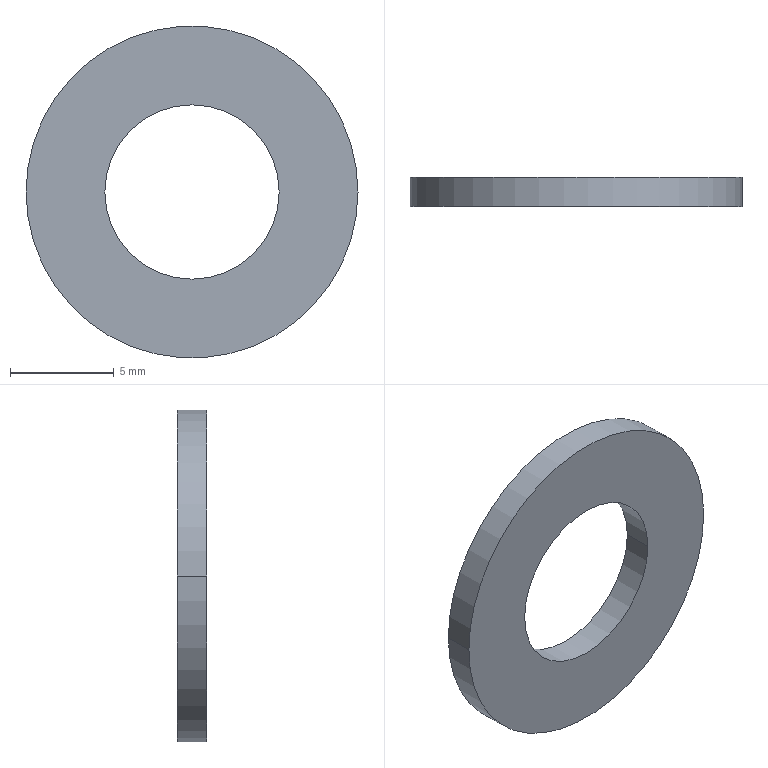Component | SolidWorks | FlatWasher_8-1 | 1 solid | 6 faces | box 16 x 1.4 x 16 mm | volume 204 mm3 | cylinder 4 | plane 2 | commonest cylinder face diameters 8.4 x2 16 x2 | material Plain Carbon Steel
build123d program:
from build123d import *

# Parameters (mm, degrees)
SKETCH1_R           = 8
SKETCH1_R_2         = 4.2
BOSS_EXTRUDE1_DEPTH = 1.4


with BuildPart() as part:
    # Sketch1 → Boss-Extrude1 (new body)
    with BuildSketch(Plane.XY):
        Circle(SKETCH1_R)
        Circle(SKETCH1_R_2, mode=Mode.SUBTRACT)
    extrude(amount=BOSS_EXTRUDE1_DEPTH)


solid = part.part

# Placed as in the assembly
solid = solid.moved(Location((29.475, -68.5, 229.781), (90, 0, 0)))
STEP:
#1=CARTESIAN_POINT('',(0.9951,-2.752,9.046));
#2=VERTEX_POINT('',#1);
#3=CARTESIAN_POINT('',(1.326,-2.752,9.046));
#4=VERTEX_POINT('',#3);
#5=CARTESIAN_POINT('',(1.16,-2.752,9.046));
#6=DIRECTION('',(0.,-1.,0.));
#7=DIRECTION('',(1.,0.,0.));
#8=AXIS2_PLACEMENT_3D('',#5,#6,#7);
#9=CIRCLE('',#8,0.1654);
#10=EDGE_CURVE('',#2,#4,#9,.T.);
#11=ORIENTED_EDGE('',*,*,#10,.T.);
#12=CARTESIAN_POINT('',(1.326,-2.697,9.046));
#13=VERTEX_POINT('',#12);
#14=CARTESIAN_POINT('',(1.326,-2.752,9.046));
#15=DIRECTION('',(-0.,1.,-0.));
#16=VECTOR('',#15,39.37);
#17=LINE('',#14,#16);
#18=EDGE_CURVE('',#4,#13,#17,.T.);
#19=ORIENTED_EDGE('',*,*,#18,.T.);
#20=CARTESIAN_POINT('',(0.9951,-2.697,9.046));
#21=VERTEX_POINT('',#20);
#22=CARTESIAN_POINT('',(1.16,-2.697,9.046));
#23=DIRECTION('',(0.,-1.,0.));
#24=DIRECTION('',(1.,0.,0.));
#25=AXIS2_PLACEMENT_3D('',#22,#23,#24);
#26=CIRCLE('',#25,0.1654);
#27=EDGE_CURVE('',#21,#13,#26,.T.);
#28=ORIENTED_EDGE('',*,*,#27,.F.);
#29=CARTESIAN_POINT('',(0.9951,-2.752,9.046));
#30=DIRECTION('',(-0.,1.,-0.));
#31=VECTOR('',#30,39.37);
#32=LINE('',#29,#31);
#33=EDGE_CURVE('',#2,#21,#32,.T.);
#34=ORIENTED_EDGE('',*,*,#33,.F.);
#35=EDGE_LOOP('',(#11,#19,#28,#34));
#36=FACE_OUTER_BOUND('',#35,.T.);
#37=CARTESIAN_POINT('',(1.16,-2.752,9.046));
#38=DIRECTION('',(-0.,1.,-0.));
#39=DIRECTION('',(-1.,0.,0.));
#40=AXIS2_PLACEMENT_3D('',#37,#38,#39);
#41=CYLINDRICAL_SURFACE('',#40,0.1654);
#42=ADVANCED_FACE('',(#36),#41,.F.);
#43=CARTESIAN_POINT('',(1.475,-2.752,9.046));
#44=VERTEX_POINT('',#43);
#45=CARTESIAN_POINT('',(0.8455,-2.752,9.046));
#46=VERTEX_POINT('',#45);
#47=CARTESIAN_POINT('',(1.16,-2.752,9.046));
#48=DIRECTION('',(0.,-1.,0.));
#49=DIRECTION('',(1.,0.,0.));
#50=AXIS2_PLACEMENT_3D('',#47,#48,#49);
#51=CIRCLE('',#50,0.315);
#52=EDGE_CURVE('',#44,#46,#51,.T.);
#53=ORIENTED_EDGE('',*,*,#52,.F.);
#54=CARTESIAN_POINT('',(1.475,-2.697,9.046));
#55=VERTEX_POINT('',#54);
#56=CARTESIAN_POINT('',(1.475,-2.752,9.046));
#57=DIRECTION('',(-0.,1.,-0.));
#58=VECTOR('',#57,39.37);
#59=LINE('',#56,#58);
#60=EDGE_CURVE('',#44,#55,#59,.T.);
#61=ORIENTED_EDGE('',*,*,#60,.T.);
#62=CARTESIAN_POINT('',(0.8455,-2.697,9.046));
#63=VERTEX_POINT('',#62);
#64=CARTESIAN_POINT('',(1.16,-2.697,9.046));
#65=DIRECTION('',(0.,-1.,0.));
#66=DIRECTION('',(1.,0.,0.));
#67=AXIS2_PLACEMENT_3D('',#64,#65,#66);
#68=CIRCLE('',#67,0.315);
#69=EDGE_CURVE('',#55,#63,#68,.T.);
#70=ORIENTED_EDGE('',*,*,#69,.T.);
#71=CARTESIAN_POINT('',(0.8455,-2.752,9.046));
#72=DIRECTION('',(-0.,1.,-0.));
#73=VECTOR('',#72,39.37);
#74=LINE('',#71,#73);
#75=EDGE_CURVE('',#46,#63,#74,.T.);
#76=ORIENTED_EDGE('',*,*,#75,.F.);
#77=EDGE_LOOP('',(#53,#61,#70,#76));
#78=FACE_OUTER_BOUND('',#77,.T.);
#79=CARTESIAN_POINT('',(1.16,-2.752,9.046));
#80=DIRECTION('',(-0.,1.,-0.));
#81=DIRECTION('',(-1.,0.,0.));
#82=AXIS2_PLACEMENT_3D('',#79,#80,#81);
#83=CYLINDRICAL_SURFACE('',#82,0.315);
#84=ADVANCED_FACE('',(#78),#83,.T.);
#85=CARTESIAN_POINT('',(1.16,-2.752,9.046));
#86=DIRECTION('',(0.,-1.,0.));
#87=DIRECTION('',(1.,0.,0.));
#88=AXIS2_PLACEMENT_3D('',#85,#86,#87);
#89=CIRCLE('',#88,0.315);
#90=EDGE_CURVE('',#46,#44,#89,.T.);
#91=ORIENTED_EDGE('',*,*,#90,.T.);
#92=ORIENTED_EDGE('',*,*,#52,.T.);
#93=EDGE_LOOP('',(#91,#92));
#94=FACE_OUTER_BOUND('',#93,.T.);
#95=ORIENTED_EDGE('',*,*,#10,.F.);
#96=CARTESIAN_POINT('',(1.16,-2.752,9.046));
#97=DIRECTION('',(0.,-1.,0.));
#98=DIRECTION('',(1.,0.,0.));
#99=AXIS2_PLACEMENT_3D('',#96,#97,#98);
#100=CIRCLE('',#99,0.1654);
#101=EDGE_CURVE('',#4,#2,#100,.T.);
#102=ORIENTED_EDGE('',*,*,#101,.F.);
#103=EDGE_LOOP('',(#95,#102));
#104=FACE_BOUND('',#103,.T.);
#105=CARTESIAN_POINT('',(1.16,-2.752,9.046));
#106=DIRECTION('',(0.,-1.,0.));
#107=DIRECTION('',(1.,0.,-0.));
#108=AXIS2_PLACEMENT_3D('',#105,#106,#107);
#109=PLANE('',#108);
#110=ADVANCED_FACE('',(#94,#104),#109,.T.);
#111=CARTESIAN_POINT('',(1.16,-2.697,9.046));
#112=DIRECTION('',(0.,-1.,0.));
#113=DIRECTION('',(1.,0.,0.));
#114=AXIS2_PLACEMENT_3D('',#111,#112,#113);
#115=CIRCLE('',#114,0.315);
#116=EDGE_CURVE('',#63,#55,#115,.T.);
#117=ORIENTED_EDGE('',*,*,#116,.F.);
#118=ORIENTED_EDGE('',*,*,#69,.F.);
#119=EDGE_LOOP('',(#117,#118));
#120=FACE_OUTER_BOUND('',#119,.T.);
#121=ORIENTED_EDGE('',*,*,#27,.T.);
#122=CARTESIAN_POINT('',(1.16,-2.697,9.046));
#123=DIRECTION('',(0.,-1.,0.));
#124=DIRECTION('',(1.,0.,0.));
#125=AXIS2_PLACEMENT_3D('',#122,#123,#124);
#126=CIRCLE('',#125,0.1654);
#127=EDGE_CURVE('',#13,#21,#126,.T.);
#128=ORIENTED_EDGE('',*,*,#127,.T.);
#129=EDGE_LOOP('',(#121,#128));
#130=FACE_BOUND('',#129,.T.);
#131=CARTESIAN_POINT('',(1.16,-2.697,9.046));
#132=DIRECTION('',(0.,-1.,0.));
#133=DIRECTION('',(1.,0.,-0.));
#134=AXIS2_PLACEMENT_3D('',#131,#132,#133);
#135=PLANE('',#134);
#136=ADVANCED_FACE('',(#120,#130),#135,.F.);
#137=ORIENTED_EDGE('',*,*,#60,.F.);
#138=ORIENTED_EDGE('',*,*,#90,.F.);
#139=ORIENTED_EDGE('',*,*,#75,.T.);
#140=ORIENTED_EDGE('',*,*,#116,.T.);
#141=EDGE_LOOP('',(#137,#138,#139,#140));
#142=FACE_OUTER_BOUND('',#141,.T.);
#143=CARTESIAN_POINT('',(1.16,-2.752,9.046));
#144=DIRECTION('',(-0.,1.,-0.));
#145=DIRECTION('',(-1.,0.,0.));
#146=AXIS2_PLACEMENT_3D('',#143,#144,#145);
#147=CYLINDRICAL_SURFACE('',#146,0.315);
#148=ADVANCED_FACE('',(#142),#147,.T.);
#149=ORIENTED_EDGE('',*,*,#18,.F.);
#150=ORIENTED_EDGE('',*,*,#101,.T.);
#151=ORIENTED_EDGE('',*,*,#33,.T.);
#152=ORIENTED_EDGE('',*,*,#127,.F.);
#153=EDGE_LOOP('',(#149,#150,#151,#152));
#154=FACE_OUTER_BOUND('',#153,.T.);
#155=CARTESIAN_POINT('',(1.16,-2.752,9.046));
#156=DIRECTION('',(-0.,1.,-0.));
#157=DIRECTION('',(-1.,0.,0.));
#158=AXIS2_PLACEMENT_3D('',#155,#156,#157);
#159=CYLINDRICAL_SURFACE('',#158,0.1654);
#160=ADVANCED_FACE('',(#154),#159,.F.);
#161=CLOSED_SHELL('',(#42,#84,#110,#136,#148,#160));
#162=MANIFOLD_SOLID_BREP('',#161);
#163=CARTESIAN_POINT('',(0.,0.,0.));
#164=DIRECTION('',(0.,0.,1.));
#165=DIRECTION('',(1.,0.,0.));
#166=AXIS2_PLACEMENT_3D('',#163,#164,#165);
#167=(LENGTH_UNIT()NAMED_UNIT(*)SI_UNIT($,.METRE.));
#168=LENGTH_MEASURE_WITH_UNIT(LENGTH_MEASURE(0.0254),#167);
#169=DIMENSIONAL_EXPONENTS(1.,0.,0.,0.,0.,0.,0.);
#170=(CONVERSION_BASED_UNIT('',#168)LENGTH_UNIT()NAMED_UNIT(#169));
#171=UNCERTAINTY_MEASURE_WITH_UNIT(LENGTH_MEASURE(0.00001),#170,'','');
#172=(NAMED_UNIT(*)PLANE_ANGLE_UNIT()SI_UNIT($,.RADIAN.));
#173=(NAMED_UNIT(*)SI_UNIT($,.STERADIAN.)SOLID_ANGLE_UNIT());
#174=(GEOMETRIC_REPRESENTATION_CONTEXT(3)GLOBAL_UNCERTAINTY_ASSIGNED_CONTEXT((#171))GLOBAL_UNIT_ASSIGNED_CONTEXT((#170,#172,#173))REPRESENTATION_CONTEXT('',''));
#175=ADVANCED_BREP_SHAPE_REPRESENTATION('',(#162,#166),#174);
#176=COLOUR_RGB('',0.7922,0.8196,0.9333);
#177=FILL_AREA_STYLE_COLOUR('',#176);
#178=FILL_AREA_STYLE('',(#177));
#179=SURFACE_STYLE_FILL_AREA(#178);
#180=SURFACE_SIDE_STYLE('',(#179));
#181=SURFACE_STYLE_USAGE(.BOTH.,#180);
#182=PRESENTATION_STYLE_ASSIGNMENT((#181));
#183=STYLED_ITEM('',(#182),#162);
#184=(LENGTH_UNIT()NAMED_UNIT(*)SI_UNIT($,.METRE.));
#185=LENGTH_MEASURE_WITH_UNIT(LENGTH_MEASURE(0.0254),#184);
#186=DIMENSIONAL_EXPONENTS(1.,0.,0.,0.,0.,0.,0.);
#187=(CONVERSION_BASED_UNIT('',#185)LENGTH_UNIT()NAMED_UNIT(#186));
#188=UNCERTAINTY_MEASURE_WITH_UNIT(LENGTH_MEASURE(0.00001),#187,'','');
#189=(NAMED_UNIT(*)PLANE_ANGLE_UNIT()SI_UNIT($,.RADIAN.));
#190=(NAMED_UNIT(*)SI_UNIT($,.STERADIAN.)SOLID_ANGLE_UNIT());
#191=(GEOMETRIC_REPRESENTATION_CONTEXT(3)GLOBAL_UNCERTAINTY_ASSIGNED_CONTEXT((#188))GLOBAL_UNIT_ASSIGNED_CONTEXT((#187,#189,#190))REPRESENTATION_CONTEXT('',''));
#192=MECHANICAL_DESIGN_GEOMETRIC_PRESENTATION_REPRESENTATION('',(#183),#191);
#193=PRESENTATION_LAYER_ASSIGNMENT('','',(#183));